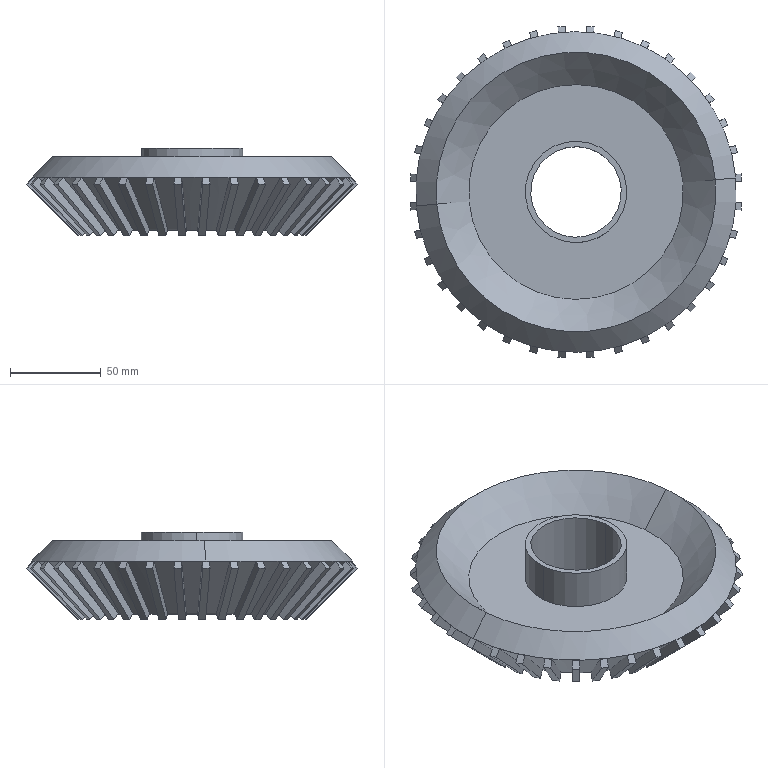Component | SolidWorks | BevelGear-1 | 1 solid | 198 faces | volume 405470 mm3 | plane 184 | cone 8 | cylinder 6 | commonest cylinder face diameters 56 x4 50 x2